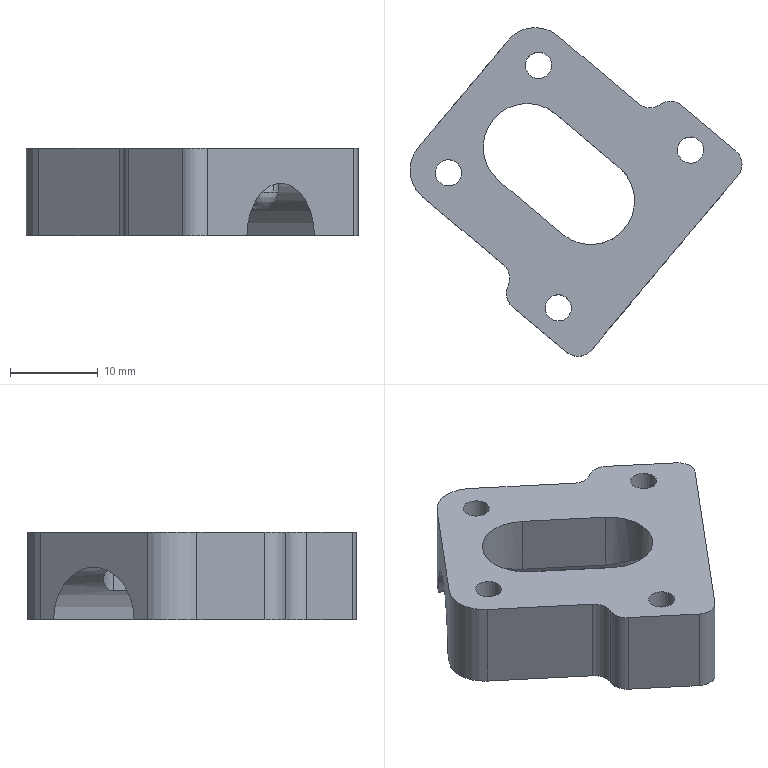Component | SolidWorks | UpperAndLowerPlateConnection-3 | 1 solid | 34 faces | box 37.88 x 37.51 x 10 mm | volume 5068 mm3 | cylinder 22 | plane 11 | sphere 1 | commonest cylinder face diameters 4 x8 3 x8 10 x3 8 x2 12 x1
build123d program:
from build123d import *

# Parameters (mm, degrees)
SKETCH2_R           = 1.5
BOSS_EXTRUDE1_DEPTH = 10
SKETCH3_R           = 6
CUT_EXTRUDE1_DEPTH  = 34
CUT_EXTRUDE2_DEPTH  = 34
SKETCH5_R           = 2
BOSS_EXTRUDE2_DEPTH = 5
DOME1_FACE_RADIUS   = 2
DOME1_HEIGHT        = 2


with BuildPart() as part:
    # Sketch2 → Boss-Extrude1 (new body)
    with BuildSketch(Plane(origin=(0, 0, 0), x_dir=(1, 0, 0), z_dir=(0, 1, 0))):
        with BuildLine():
            Line((-13, 30), (13, 30))
            ThreePointArc((13, 30), (14.414, 29.414), (15, 28))
            Line((15, 28), (15, 19.936))
            ThreePointArc((15, 19.936), (14.581, 18.712), (13.5, 18))
            ThreePointArc((13.5, 18), (12.419, 17.288), (12, 16.064))
            Line((12, 16.064), (12, 4))
            ThreePointArc((12, 4), (10.828, 1.172), (8, 0))
            Line((8, 0), (-8, 0))
            ThreePointArc((-8, 0), (-10.828, 1.172), (-12, 4))
            Line((-12, 4), (-12, 16.064))
            ThreePointArc((-12, 16.064), (-12.419, 17.288), (-13.5, 18))
            ThreePointArc((-13.5, 18), (-14.581, 18.712), (-15, 19.936))
            Line((-15, 19.936), (-15, 28))
            ThreePointArc((-15, 28), (-14.414, 29.414), (-13, 30))
        make_face()
        with Locations(Location((11.75, 24, 0), (0, 0, 270))):
            Circle(SKETCH2_R, mode=Mode.SUBTRACT)
        with Locations(Location((8, 4.5, 0), (0, 0, 270))):
            Circle(SKETCH2_R, mode=Mode.SUBTRACT)
        with Locations(Location((-8, 4.5, 0), (0, 0, 90))):
            Circle(SKETCH2_R, mode=Mode.SUBTRACT)
        with Locations(Location((-11.75, 24, 0), (0, 0, 90))):
            Circle(SKETCH2_R, mode=Mode.SUBTRACT)
    extrude(amount=BOSS_EXTRUDE1_DEPTH)

    # Sketch3 → Cut-Extrude1 (cut)
    with BuildSketch(Plane.XY):
        Circle(SKETCH3_R)
    extrude(amount=-CUT_EXTRUDE1_DEPTH, mode=Mode.SUBTRACT)

    # Sketch4 → Cut-Extrude2 (cut)
    with BuildSketch(Plane(origin=(0, 10, 0), x_dir=(1, 0, 0), z_dir=(0, 1, 0))):
        with BuildLine():
            Line((5, 19), (5, 9.5))
            ThreePointArc((5, 9.5), (0, 4.5), (-5, 9.5))
            Line((-5, 9.5), (-5, 19))
            ThreePointArc((-5, 19), (0, 24), (5, 19))
        make_face()
    extrude(amount=-CUT_EXTRUDE2_DEPTH, mode=Mode.SUBTRACT)

    # Sketch5 → Boss-Extrude2 (add)
    with BuildSketch(Plane(origin=(0, 10, 0), x_dir=(1, 0, 0), z_dir=(0, 1, 0))):
        with Locations(Location((0, 27, 0), (0, 0, 270))):
            Circle(SKETCH5_R)
    extrude(amount=-BOSS_EXTRUDE2_DEPTH)

    # Dome1: a dome of height H over a round flat face of radius A is a cap of a sphere of radius (A * A + H * H) / (2 * H)
    dome1_r = (DOME1_FACE_RADIUS * DOME1_FACE_RADIUS + DOME1_HEIGHT * DOME1_HEIGHT) / (2 * DOME1_HEIGHT)
    dome1_base = Plane((0, 5, -27), z_dir=(0, -1, 0))
    with Locations(dome1_base.offset(DOME1_HEIGHT - dome1_r)):
        dome1_ball = Sphere(dome1_r, mode=Mode.PRIVATE)
    add(split(dome1_ball, bisect_by=dome1_base, keep=Keep.TOP, mode=Mode.PRIVATE))


solid = part.part

# Placed as in the assembly
solid = solid.moved(Location((4.787, -44.148, 1027.6), (-90, -50, -180)))